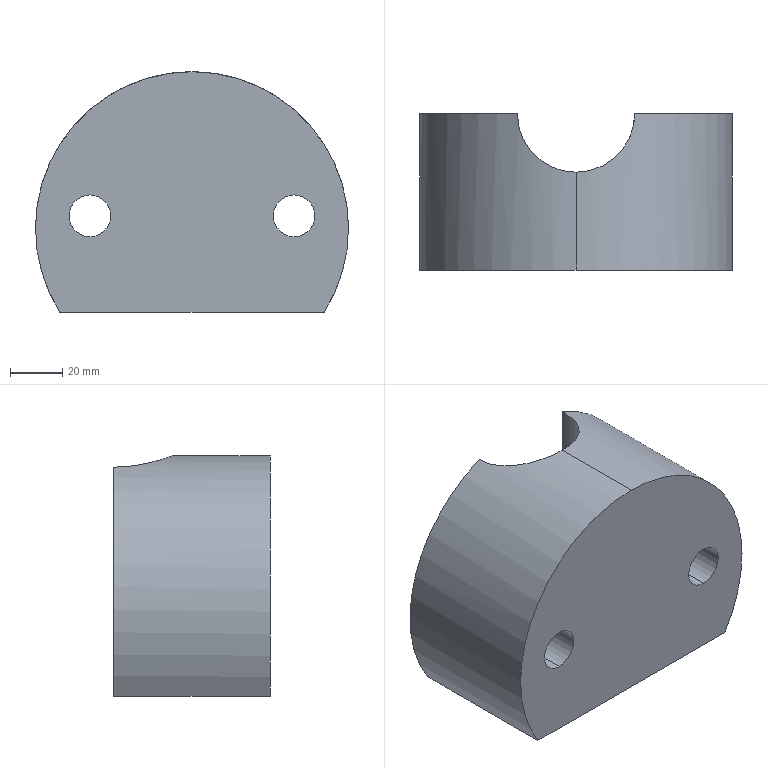Component | SolidWorks | PressureBlock-1 | 1 solid | 12 faces | box 120 x 60 x 92.21 mm | volume 462926 mm3 | cylinder 8 | plane 4 | commonest cylinder face diameters 16 x4 45 x2 120 x2
build123d program:
from build123d import *

# Parameters (mm, degrees)
BOSS_EXTRUDE1_DEPTH        = 60
M39_CLEARANCE_HOLE1_D      = 45
F_16_0_16_DIAMETER_HOLE1_D = 16


with BuildPart() as part:
    # Sketch1 → Boss-Extrude1 (new body)
    with BuildSketch(Plane.XY.offset(60)):
        with BuildLine():
            Line((-37.256, 16.825), (-37.256, -84.417))
            ThreePointArc((-37.256, -84.417), (54.954, -33.796), (-37.256, 16.825))
        make_face()
    extrude(amount=-BOSS_EXTRUDE1_DEPTH)

    # M39 Clearance Hole1 (through all)
    with Locations(Plane.ZY.offset(37.256)):
        with Locations((0, -33.796)):
            Hole(M39_CLEARANCE_HOLE1_D / 2)

    # 16.0 _16_ Diameter Hole1 (through all)
    with Locations(Plane(origin=(0, 0, 0), x_dir=(-1, 0, 0), z_dir=(0, 0, -1))):
        with Locations((0.3007, -72.931), (0.3007, 5.34)):
            Hole(F_16_0_16_DIAMETER_HOLE1_D / 2)


solid = part.part

# Placed as in the assembly
solid = solid.moved(Location((-536.128, 847.548, 422.709), (90, 0, 90)))
STEP:
#1=COLOUR_RGB('',0.7922,0.8196,0.9333);
#2=FILL_AREA_STYLE_COLOUR('',#1);
#3=FILL_AREA_STYLE('',(#2));
#4=SURFACE_STYLE_FILL_AREA(#3);
#5=SURFACE_SIDE_STYLE('',(#4));
#6=SURFACE_STYLE_USAGE(.BOTH.,#5);
#7=PRESENTATION_STYLE_ASSIGNMENT((#6));
#8=CARTESIAN_POINT('',(-18.236,31.006,16.945));
#9=VERTEX_POINT('',#8);
#10=CARTESIAN_POINT('',(-18.236,31.006,16.315));
#11=VERTEX_POINT('',#10);
#12=CARTESIAN_POINT('',(-18.236,31.006,16.63));
#13=DIRECTION('',(0.,1.,0.));
#14=DIRECTION('',(0.,0.,-1.));
#15=AXIS2_PLACEMENT_3D('',#12,#13,#14);
#16=CIRCLE('',#15,0.315);
#17=EDGE_CURVE('',#9,#11,#16,.T.);
#18=ORIENTED_EDGE('',*,*,#17,.F.);
#19=CARTESIAN_POINT('',(-18.236,33.368,16.945));
#20=VERTEX_POINT('',#19);
#21=CARTESIAN_POINT('',(-18.236,33.368,16.945));
#22=DIRECTION('',(0.,1.,0.));
#23=VECTOR('',#22,39.37);
#24=LINE('',#21,#23);
#25=EDGE_CURVE('',#9,#20,#24,.T.);
#26=ORIENTED_EDGE('',*,*,#25,.T.);
#27=CARTESIAN_POINT('',(-18.236,33.368,16.315));
#28=VERTEX_POINT('',#27);
#29=CARTESIAN_POINT('',(-18.236,33.368,16.63));
#30=DIRECTION('',(0.,1.,0.));
#31=DIRECTION('',(0.,0.,-1.));
#32=AXIS2_PLACEMENT_3D('',#29,#30,#31);
#33=CIRCLE('',#32,0.315);
#34=EDGE_CURVE('',#20,#28,#33,.T.);
#35=ORIENTED_EDGE('',*,*,#34,.T.);
#36=CARTESIAN_POINT('',(-18.236,33.368,16.315));
#37=DIRECTION('',(0.,1.,0.));
#38=VECTOR('',#37,39.37);
#39=LINE('',#36,#38);
#40=EDGE_CURVE('',#11,#28,#39,.T.);
#41=ORIENTED_EDGE('',*,*,#40,.F.);
#42=EDGE_LOOP('',(#18,#26,#35,#41));
#43=FACE_OUTER_BOUND('',#42,.T.);
#44=CARTESIAN_POINT('',(-18.236,33.368,16.63));
#45=DIRECTION('',(0.,1.,0.));
#46=DIRECTION('',(0.,0.,-1.));
#47=AXIS2_PLACEMENT_3D('',#44,#45,#46);
#48=CYLINDRICAL_SURFACE('',#47,0.315);
#49=ADVANCED_FACE('',(#43),#48,.F.);
#50=CARTESIAN_POINT('',(-21.318,31.006,16.945));
#51=VERTEX_POINT('',#50);
#52=CARTESIAN_POINT('',(-21.318,31.006,16.315));
#53=VERTEX_POINT('',#52);
#54=CARTESIAN_POINT('',(-21.318,31.006,16.63));
#55=DIRECTION('',(0.,1.,0.));
#56=DIRECTION('',(0.,0.,-1.));
#57=AXIS2_PLACEMENT_3D('',#54,#55,#56);
#58=CIRCLE('',#57,0.315);
#59=EDGE_CURVE('',#51,#53,#58,.T.);
#60=ORIENTED_EDGE('',*,*,#59,.F.);
#61=CARTESIAN_POINT('',(-21.318,33.368,16.945));
#62=VERTEX_POINT('',#61);
#63=CARTESIAN_POINT('',(-21.318,33.368,16.945));
#64=DIRECTION('',(0.,1.,0.));
#65=VECTOR('',#64,39.37);
#66=LINE('',#63,#65);
#67=EDGE_CURVE('',#51,#62,#66,.T.);
#68=ORIENTED_EDGE('',*,*,#67,.T.);
#69=CARTESIAN_POINT('',(-21.318,33.368,16.315));
#70=VERTEX_POINT('',#69);
#71=CARTESIAN_POINT('',(-21.318,33.368,16.63));
#72=DIRECTION('',(0.,1.,0.));
#73=DIRECTION('',(0.,0.,-1.));
#74=AXIS2_PLACEMENT_3D('',#71,#72,#73);
#75=CIRCLE('',#74,0.315);
#76=EDGE_CURVE('',#62,#70,#75,.T.);
#77=ORIENTED_EDGE('',*,*,#76,.T.);
#78=CARTESIAN_POINT('',(-21.318,33.368,16.315));
#79=DIRECTION('',(0.,1.,0.));
#80=VECTOR('',#79,39.37);
#81=LINE('',#78,#80);
#82=EDGE_CURVE('',#53,#70,#81,.T.);
#83=ORIENTED_EDGE('',*,*,#82,.F.);
#84=EDGE_LOOP('',(#60,#68,#77,#83));
#85=FACE_OUTER_BOUND('',#84,.T.);
#86=CARTESIAN_POINT('',(-21.318,33.368,16.63));
#87=DIRECTION('',(0.,1.,0.));
#88=DIRECTION('',(0.,0.,-1.));
#89=AXIS2_PLACEMENT_3D('',#86,#87,#88);
#90=CYLINDRICAL_SURFACE('',#89,0.315);
#91=ADVANCED_FACE('',(#85),#90,.F.);
#92=CARTESIAN_POINT('',(-20.663,33.368,18.633));
#93=VERTEX_POINT('',#92);
#94=CARTESIAN_POINT('',(-19.777,32.482,18.806));
#95=VERTEX_POINT('',#94);
#96=CARTESIAN_POINT('',(-20.663,33.368,18.633));
#97=CARTESIAN_POINT('',(-20.663,33.309,18.633));
#98=CARTESIAN_POINT('',(-20.657,33.251,18.636));
#99=CARTESIAN_POINT('',(-20.64,33.166,18.642));
#100=CARTESIAN_POINT('',(-20.633,33.137,18.645));
#101=CARTESIAN_POINT('',(-20.62,33.095,18.65));
#102=CARTESIAN_POINT('',(-20.615,33.082,18.652));
#103=CARTESIAN_POINT('',(-20.605,33.054,18.656));
#104=CARTESIAN_POINT('',(-20.6,33.041,18.658));
#105=CARTESIAN_POINT('',(-20.572,32.974,18.668));
#106=CARTESIAN_POINT('',(-20.545,32.923,18.678));
#107=CARTESIAN_POINT('',(-20.497,32.851,18.693));
#108=CARTESIAN_POINT('',(-20.479,32.828,18.699));
#109=CARTESIAN_POINT('',(-20.443,32.783,18.71));
#110=CARTESIAN_POINT('',(-20.424,32.762,18.715));
#111=CARTESIAN_POINT('',(-20.383,32.722,18.727));
#112=CARTESIAN_POINT('',(-20.362,32.702,18.732));
#113=CARTESIAN_POINT('',(-20.318,32.666,18.743));
#114=CARTESIAN_POINT('',(-20.295,32.649,18.748));
#115=CARTESIAN_POINT('',(-20.222,32.6,18.764));
#116=CARTESIAN_POINT('',(-20.172,32.573,18.773));
#117=CARTESIAN_POINT('',(-20.092,32.54,18.785));
#118=CARTESIAN_POINT('',(-20.065,32.53,18.788));
#119=CARTESIAN_POINT('',(-20.009,32.513,18.794));
#120=CARTESIAN_POINT('',(-19.98,32.505,18.797));
#121=CARTESIAN_POINT('',(-19.894,32.488,18.803));
#122=CARTESIAN_POINT('',(-19.836,32.482,18.806));
#123=CARTESIAN_POINT('',(-19.777,32.482,18.806));
#124=B_SPLINE_CURVE_WITH_KNOTS('',3,(#96,#97,#98,#99,#100,#101,#102,#103,#104,#105,#106,#107,#108,#109,#110,#111,#112,#113,#114,#115,#116,#117,#118,#119,#120,#121,#122,#123),.UNSPECIFIED.,.F.,.F.,(4,2,2,2,2,2,2,2,2,2,2,2,2,4),(-0.03548,-0.03104,-0.02883,-0.02772,-0.02661,-0.02217,-0.01996,-0.01774,-0.01552,-0.0133,-0.00887,-0.006652,-0.004435,-0.),.UNSPECIFIED.);
#125=EDGE_CURVE('',#93,#95,#124,.T.);
#126=ORIENTED_EDGE('',*,*,#125,.T.);
#127=CARTESIAN_POINT('',(-19.777,32.482,15.175));
#128=VERTEX_POINT('',#127);
#129=CARTESIAN_POINT('',(-19.777,32.482,15.175));
#130=DIRECTION('',(0.,0.,-1.));
#131=VECTOR('',#130,39.37);
#132=LINE('',#129,#131);
#133=EDGE_CURVE('',#95,#128,#132,.T.);
#134=ORIENTED_EDGE('',*,*,#133,.T.);
#135=CARTESIAN_POINT('',(-20.663,33.368,15.175));
#136=VERTEX_POINT('',#135);
#137=CARTESIAN_POINT('',(-19.777,33.368,15.175));
#138=DIRECTION('',(0.,0.,-1.));
#139=DIRECTION('',(0.,-1.,0.));
#140=AXIS2_PLACEMENT_3D('',#137,#138,#139);
#141=CIRCLE('',#140,0.8858);
#142=EDGE_CURVE('',#128,#136,#141,.T.);
#143=ORIENTED_EDGE('',*,*,#142,.T.);
#144=CARTESIAN_POINT('',(-20.663,33.368,15.175));
#145=DIRECTION('',(0.,0.,-1.));
#146=VECTOR('',#145,39.37);
#147=LINE('',#144,#146);
#148=EDGE_CURVE('',#93,#136,#147,.T.);
#149=ORIENTED_EDGE('',*,*,#148,.F.);
#150=EDGE_LOOP('',(#126,#134,#143,#149));
#151=FACE_OUTER_BOUND('',#150,.T.);
#152=CARTESIAN_POINT('',(-19.777,33.368,15.175));
#153=DIRECTION('',(0.,0.,-1.));
#154=DIRECTION('',(0.,-1.,0.));
#155=AXIS2_PLACEMENT_3D('',#152,#153,#154);
#156=CYLINDRICAL_SURFACE('',#155,0.8858);
#157=ADVANCED_FACE('',(#151),#156,.F.);
#158=CARTESIAN_POINT('',(-18.891,33.368,18.633));
#159=VERTEX_POINT('',#158);
#160=CARTESIAN_POINT('',(-19.777,32.482,18.806));
#161=CARTESIAN_POINT('',(-19.718,32.482,18.806));
#162=CARTESIAN_POINT('',(-19.66,32.488,18.803));
#163=CARTESIAN_POINT('',(-19.574,32.505,18.797));
#164=CARTESIAN_POINT('',(-19.546,32.512,18.795));
#165=CARTESIAN_POINT('',(-19.504,32.525,18.79));
#166=CARTESIAN_POINT('',(-19.49,32.53,18.788));
#167=CARTESIAN_POINT('',(-19.463,32.54,18.785));
#168=CARTESIAN_POINT('',(-19.449,32.545,18.783));
#169=CARTESIAN_POINT('',(-19.382,32.573,18.773));
#170=CARTESIAN_POINT('',(-19.332,32.6,18.764));
#171=CARTESIAN_POINT('',(-19.26,32.648,18.748));
#172=CARTESIAN_POINT('',(-19.236,32.666,18.743));
#173=CARTESIAN_POINT('',(-19.192,32.702,18.732));
#174=CARTESIAN_POINT('',(-19.171,32.721,18.727));
#175=CARTESIAN_POINT('',(-19.11,32.782,18.71));
#176=CARTESIAN_POINT('',(-19.073,32.826,18.699));
#177=CARTESIAN_POINT('',(-19.009,32.923,18.678));
#178=CARTESIAN_POINT('',(-18.982,32.973,18.668));
#179=CARTESIAN_POINT('',(-18.948,33.053,18.656));
#180=CARTESIAN_POINT('',(-18.939,33.08,18.652));
#181=CARTESIAN_POINT('',(-18.921,33.136,18.645));
#182=CARTESIAN_POINT('',(-18.914,33.165,18.643));
#183=CARTESIAN_POINT('',(-18.897,33.251,18.636));
#184=CARTESIAN_POINT('',(-18.891,33.309,18.633));
#185=CARTESIAN_POINT('',(-18.891,33.368,18.633));
#186=B_SPLINE_CURVE_WITH_KNOTS('',3,(#160,#161,#162,#163,#164,#165,#166,#167,#168,#169,#170,#171,#172,#173,#174,#175,#176,#177,#178,#179,#180,#181,#182,#183,#184,#185),.UNSPECIFIED.,.F.,.F.,(4,2,2,2,2,2,2,2,2,2,2,2,4),(-0.,0.004435,0.006652,0.007761,0.00887,0.0133,0.01552,0.01774,0.02217,0.02661,0.02883,0.03104,0.03548),.UNSPECIFIED.);
#187=EDGE_CURVE('',#95,#159,#186,.T.);
#188=ORIENTED_EDGE('',*,*,#187,.F.);
#189=CARTESIAN_POINT('',(-19.777,31.006,18.806));
#190=VERTEX_POINT('',#189);
#191=CARTESIAN_POINT('',(-19.777,33.368,18.806));
#192=DIRECTION('',(0.,-1.,0.));
#193=VECTOR('',#192,39.37);
#194=LINE('',#191,#193);
#195=EDGE_CURVE('',#95,#190,#194,.T.);
#196=ORIENTED_EDGE('',*,*,#195,.T.);
#197=CARTESIAN_POINT('',(-17.784,31.006,15.175));
#198=VERTEX_POINT('',#197);
#199=CARTESIAN_POINT('',(-19.777,31.006,16.443));
#200=DIRECTION('',(0.,-1.,0.));
#201=DIRECTION('',(0.,0.,1.));
#202=AXIS2_PLACEMENT_3D('',#199,#200,#201);
#203=CIRCLE('',#202,2.362);
#204=EDGE_CURVE('',#198,#190,#203,.T.);
#205=ORIENTED_EDGE('',*,*,#204,.F.);
#206=CARTESIAN_POINT('',(-17.784,33.368,15.175));
#207=VERTEX_POINT('',#206);
#208=CARTESIAN_POINT('',(-17.784,33.368,15.175));
#209=DIRECTION('',(0.,-1.,0.));
#210=VECTOR('',#209,39.37);
#211=LINE('',#208,#210);
#212=EDGE_CURVE('',#207,#198,#211,.T.);
#213=ORIENTED_EDGE('',*,*,#212,.F.);
#214=CARTESIAN_POINT('',(-19.777,33.368,16.443));
#215=DIRECTION('',(0.,-1.,0.));
#216=DIRECTION('',(0.,0.,1.));
#217=AXIS2_PLACEMENT_3D('',#214,#215,#216);
#218=CIRCLE('',#217,2.362);
#219=EDGE_CURVE('',#207,#159,#218,.T.);
#220=ORIENTED_EDGE('',*,*,#219,.T.);
#221=EDGE_LOOP('',(#188,#196,#205,#213,#220));
#222=FACE_OUTER_BOUND('',#221,.T.);
#223=CARTESIAN_POINT('',(-19.777,33.368,16.443));
#224=DIRECTION('',(0.,-1.,0.));
#225=DIRECTION('',(0.,0.,1.));
#226=AXIS2_PLACEMENT_3D('',#223,#224,#225);
#227=CYLINDRICAL_SURFACE('',#226,2.362);
#228=ADVANCED_FACE('',(#222),#227,.T.);
#229=ORIENTED_EDGE('',*,*,#204,.T.);
#230=CARTESIAN_POINT('',(-21.77,31.006,15.175));
#231=VERTEX_POINT('',#230);
#232=CARTESIAN_POINT('',(-19.777,31.006,16.443));
#233=DIRECTION('',(0.,-1.,0.));
#234=DIRECTION('',(0.,0.,1.));
#235=AXIS2_PLACEMENT_3D('',#232,#233,#234);
#236=CIRCLE('',#235,2.362);
#237=EDGE_CURVE('',#190,#231,#236,.T.);
#238=ORIENTED_EDGE('',*,*,#237,.T.);
#239=CARTESIAN_POINT('',(-21.77,31.006,15.175));
#240=DIRECTION('',(1.,0.,-0.));
#241=VECTOR('',#240,39.37);
#242=LINE('',#239,#241);
#243=EDGE_CURVE('',#231,#198,#242,.T.);
#244=ORIENTED_EDGE('',*,*,#243,.T.);
#245=EDGE_LOOP('',(#229,#238,#244));
#246=FACE_OUTER_BOUND('',#245,.T.);
#247=CARTESIAN_POINT('',(-21.318,31.006,16.63));
#248=DIRECTION('',(0.,1.,0.));
#249=DIRECTION('',(0.,0.,-1.));
#250=AXIS2_PLACEMENT_3D('',#247,#248,#249);
#251=CIRCLE('',#250,0.315);
#252=EDGE_CURVE('',#53,#51,#251,.T.);
#253=ORIENTED_EDGE('',*,*,#252,.T.);
#254=ORIENTED_EDGE('',*,*,#59,.T.);
#255=EDGE_LOOP('',(#253,#254));
#256=FACE_BOUND('',#255,.T.);
#257=CARTESIAN_POINT('',(-18.236,31.006,16.63));
#258=DIRECTION('',(0.,1.,0.));
#259=DIRECTION('',(0.,0.,-1.));
#260=AXIS2_PLACEMENT_3D('',#257,#258,#259);
#261=CIRCLE('',#260,0.315);
#262=EDGE_CURVE('',#11,#9,#261,.T.);
#263=ORIENTED_EDGE('',*,*,#262,.T.);
#264=ORIENTED_EDGE('',*,*,#17,.T.);
#265=EDGE_LOOP('',(#263,#264));
#266=FACE_BOUND('',#265,.T.);
#267=CARTESIAN_POINT('',(-19.777,31.006,16.443));
#268=DIRECTION('',(0.,-1.,0.));
#269=DIRECTION('',(0.,0.,1.));
#270=AXIS2_PLACEMENT_3D('',#267,#268,#269);
#271=PLANE('',#270);
#272=ADVANCED_FACE('',(#246,#256,#266),#271,.T.);
#273=CARTESIAN_POINT('',(-21.77,33.368,15.175));
#274=VERTEX_POINT('',#273);
#275=CARTESIAN_POINT('',(-19.777,33.368,16.443));
#276=DIRECTION('',(0.,-1.,0.));
#277=DIRECTION('',(0.,0.,1.));
#278=AXIS2_PLACEMENT_3D('',#275,#276,#277);
#279=CIRCLE('',#278,2.362);
#280=EDGE_CURVE('',#93,#274,#279,.T.);
#281=ORIENTED_EDGE('',*,*,#280,.F.);
#282=ORIENTED_EDGE('',*,*,#148,.T.);
#283=CARTESIAN_POINT('',(-21.77,33.368,15.175));
#284=DIRECTION('',(1.,0.,-0.));
#285=VECTOR('',#284,39.37);
#286=LINE('',#283,#285);
#287=EDGE_CURVE('',#274,#136,#286,.T.);
#288=ORIENTED_EDGE('',*,*,#287,.F.);
#289=EDGE_LOOP('',(#281,#282,#288));
#290=FACE_OUTER_BOUND('',#289,.T.);
#291=CARTESIAN_POINT('',(-21.318,33.368,16.63));
#292=DIRECTION('',(0.,1.,0.));
#293=DIRECTION('',(0.,0.,-1.));
#294=AXIS2_PLACEMENT_3D('',#291,#292,#293);
#295=CIRCLE('',#294,0.315);
#296=EDGE_CURVE('',#70,#62,#295,.T.);
#297=ORIENTED_EDGE('',*,*,#296,.F.);
#298=ORIENTED_EDGE('',*,*,#76,.F.);
#299=EDGE_LOOP('',(#297,#298));
#300=FACE_BOUND('',#299,.T.);
#301=CARTESIAN_POINT('',(-19.777,33.368,16.443));
#302=DIRECTION('',(0.,-1.,0.));
#303=DIRECTION('',(0.,0.,1.));
#304=AXIS2_PLACEMENT_3D('',#301,#302,#303);
#305=PLANE('',#304);
#306=ADVANCED_FACE('',(#290,#300),#305,.F.);
#307=ORIENTED_EDGE('',*,*,#195,.F.);
#308=ORIENTED_EDGE('',*,*,#125,.F.);
#309=ORIENTED_EDGE('',*,*,#280,.T.);
#310=CARTESIAN_POINT('',(-21.77,33.368,15.175));
#311=DIRECTION('',(0.,-1.,0.));
#312=VECTOR('',#311,39.37);
#313=LINE('',#310,#312);
#314=EDGE_CURVE('',#274,#231,#313,.T.);
#315=ORIENTED_EDGE('',*,*,#314,.T.);
#316=ORIENTED_EDGE('',*,*,#237,.F.);
#317=EDGE_LOOP('',(#307,#308,#309,#315,#316));
#318=FACE_OUTER_BOUND('',#317,.T.);
#319=CARTESIAN_POINT('',(-19.777,33.368,16.443));
#320=DIRECTION('',(0.,-1.,0.));
#321=DIRECTION('',(0.,0.,1.));
#322=AXIS2_PLACEMENT_3D('',#319,#320,#321);
#323=CYLINDRICAL_SURFACE('',#322,2.362);
#324=ADVANCED_FACE('',(#318),#323,.T.);
#325=CARTESIAN_POINT('',(-18.891,33.368,15.175));
#326=VERTEX_POINT('',#325);
#327=CARTESIAN_POINT('',(-19.777,33.368,15.175));
#328=DIRECTION('',(0.,0.,-1.));
#329=DIRECTION('',(0.,-1.,0.));
#330=AXIS2_PLACEMENT_3D('',#327,#328,#329);
#331=CIRCLE('',#330,0.8858);
#332=EDGE_CURVE('',#326,#128,#331,.T.);
#333=ORIENTED_EDGE('',*,*,#332,.F.);
#334=CARTESIAN_POINT('',(-21.77,33.368,15.175));
#335=DIRECTION('',(1.,0.,-0.));
#336=VECTOR('',#335,39.37);
#337=LINE('',#334,#336);
#338=EDGE_CURVE('',#326,#207,#337,.T.);
#339=ORIENTED_EDGE('',*,*,#338,.T.);
#340=ORIENTED_EDGE('',*,*,#212,.T.);
#341=ORIENTED_EDGE('',*,*,#243,.F.);
#342=ORIENTED_EDGE('',*,*,#314,.F.);
#343=ORIENTED_EDGE('',*,*,#287,.T.);
#344=ORIENTED_EDGE('',*,*,#142,.F.);
#345=EDGE_LOOP('',(#333,#339,#340,#341,#342,#343,#344));
#346=FACE_OUTER_BOUND('',#345,.T.);
#347=CARTESIAN_POINT('',(-21.77,33.368,15.175));
#348=DIRECTION('',(-0.,0.,-1.));
#349=DIRECTION('',(1.,0.,-0.));
#350=AXIS2_PLACEMENT_3D('',#347,#348,#349);
#351=PLANE('',#350);
#352=ADVANCED_FACE('',(#346),#351,.T.);
#353=CARTESIAN_POINT('',(-18.236,33.368,16.63));
#354=DIRECTION('',(0.,1.,0.));
#355=DIRECTION('',(0.,0.,-1.));
#356=AXIS2_PLACEMENT_3D('',#353,#354,#355);
#357=CIRCLE('',#356,0.315);
#358=EDGE_CURVE('',#28,#20,#357,.T.);
#359=ORIENTED_EDGE('',*,*,#358,.F.);
#360=ORIENTED_EDGE('',*,*,#34,.F.);
#361=EDGE_LOOP('',(#359,#360));
#362=FACE_BOUND('',#361,.T.);
#363=ORIENTED_EDGE('',*,*,#338,.F.);
#364=CARTESIAN_POINT('',(-18.891,33.368,15.175));
#365=DIRECTION('',(0.,0.,1.));
#366=VECTOR('',#365,39.37);
#367=LINE('',#364,#366);
#368=EDGE_CURVE('',#326,#159,#367,.T.);
#369=ORIENTED_EDGE('',*,*,#368,.T.);
#370=ORIENTED_EDGE('',*,*,#219,.F.);
#371=EDGE_LOOP('',(#363,#369,#370));
#372=FACE_OUTER_BOUND('',#371,.T.);
#373=CARTESIAN_POINT('',(-19.777,33.368,16.443));
#374=DIRECTION('',(0.,-1.,0.));
#375=DIRECTION('',(0.,0.,1.));
#376=AXIS2_PLACEMENT_3D('',#373,#374,#375);
#377=PLANE('',#376);
#378=ADVANCED_FACE('',(#362,#372),#377,.F.);
#379=ORIENTED_EDGE('',*,*,#133,.F.);
#380=ORIENTED_EDGE('',*,*,#187,.T.);
#381=ORIENTED_EDGE('',*,*,#368,.F.);
#382=ORIENTED_EDGE('',*,*,#332,.T.);
#383=EDGE_LOOP('',(#379,#380,#381,#382));
#384=FACE_OUTER_BOUND('',#383,.T.);
#385=CARTESIAN_POINT('',(-19.777,33.368,15.175));
#386=DIRECTION('',(0.,0.,-1.));
#387=DIRECTION('',(0.,-1.,0.));
#388=AXIS2_PLACEMENT_3D('',#385,#386,#387);
#389=CYLINDRICAL_SURFACE('',#388,0.8858);
#390=ADVANCED_FACE('',(#384),#389,.F.);
#391=ORIENTED_EDGE('',*,*,#67,.F.);
#392=ORIENTED_EDGE('',*,*,#252,.F.);
#393=ORIENTED_EDGE('',*,*,#82,.T.);
#394=ORIENTED_EDGE('',*,*,#296,.T.);
#395=EDGE_LOOP('',(#391,#392,#393,#394));
#396=FACE_OUTER_BOUND('',#395,.T.);
#397=CARTESIAN_POINT('',(-21.318,33.368,16.63));
#398=DIRECTION('',(0.,1.,0.));
#399=DIRECTION('',(0.,0.,-1.));
#400=AXIS2_PLACEMENT_3D('',#397,#398,#399);
#401=CYLINDRICAL_SURFACE('',#400,0.315);
#402=ADVANCED_FACE('',(#396),#401,.F.);
#403=ORIENTED_EDGE('',*,*,#25,.F.);
#404=ORIENTED_EDGE('',*,*,#262,.F.);
#405=ORIENTED_EDGE('',*,*,#40,.T.);
#406=ORIENTED_EDGE('',*,*,#358,.T.);
#407=EDGE_LOOP('',(#403,#404,#405,#406));
#408=FACE_OUTER_BOUND('',#407,.T.);
#409=CARTESIAN_POINT('',(-18.236,33.368,16.63));
#410=DIRECTION('',(0.,1.,0.));
#411=DIRECTION('',(0.,0.,-1.));
#412=AXIS2_PLACEMENT_3D('',#409,#410,#411);
#413=CYLINDRICAL_SURFACE('',#412,0.315);
#414=ADVANCED_FACE('',(#408),#413,.F.);
#415=CLOSED_SHELL('',(#49,#91,#157,#228,#272,#306,#324,#352,#378,#390,#402,#414));
#416=MANIFOLD_SOLID_BREP('',#415);
#417=STYLED_ITEM('',(#7),#416);
#418=(LENGTH_UNIT()NAMED_UNIT(*)SI_UNIT($,.METRE.));
#419=LENGTH_MEASURE_WITH_UNIT(LENGTH_MEASURE(0.0254),#418);
#420=DIMENSIONAL_EXPONENTS(1.,0.,0.,0.,0.,0.,0.);
#421=(CONVERSION_BASED_UNIT('',#419)LENGTH_UNIT()NAMED_UNIT(#420));
#422=UNCERTAINTY_MEASURE_WITH_UNIT(LENGTH_MEASURE(0.00001),#421,'','');
#423=(NAMED_UNIT(*)PLANE_ANGLE_UNIT()SI_UNIT($,.RADIAN.));
#424=(NAMED_UNIT(*)SI_UNIT($,.STERADIAN.)SOLID_ANGLE_UNIT());
#425=(GEOMETRIC_REPRESENTATION_CONTEXT(3)GLOBAL_UNCERTAINTY_ASSIGNED_CONTEXT((#422))GLOBAL_UNIT_ASSIGNED_CONTEXT((#421,#423,#424))REPRESENTATION_CONTEXT('',''));
#426=MECHANICAL_DESIGN_GEOMETRIC_PRESENTATION_REPRESENTATION('',(#417),#425);
#427=CARTESIAN_POINT('',(0.,0.,0.));
#428=DIRECTION('',(0.,0.,1.));
#429=DIRECTION('',(1.,0.,0.));
#430=AXIS2_PLACEMENT_3D('',#427,#428,#429);
#431=(LENGTH_UNIT()NAMED_UNIT(*)SI_UNIT($,.METRE.));
#432=LENGTH_MEASURE_WITH_UNIT(LENGTH_MEASURE(0.0254),#431);
#433=DIMENSIONAL_EXPONENTS(1.,0.,0.,0.,0.,0.,0.);
#434=(CONVERSION_BASED_UNIT('',#432)LENGTH_UNIT()NAMED_UNIT(#433));
#435=UNCERTAINTY_MEASURE_WITH_UNIT(LENGTH_MEASURE(0.00001),#434,'','');
#436=(NAMED_UNIT(*)PLANE_ANGLE_UNIT()SI_UNIT($,.RADIAN.));
#437=(NAMED_UNIT(*)SI_UNIT($,.STERADIAN.)SOLID_ANGLE_UNIT());
#438=(GEOMETRIC_REPRESENTATION_CONTEXT(3)GLOBAL_UNCERTAINTY_ASSIGNED_CONTEXT((#435))GLOBAL_UNIT_ASSIGNED_CONTEXT((#434,#436,#437))REPRESENTATION_CONTEXT('',''));
#439=ADVANCED_BREP_SHAPE_REPRESENTATION('',(#416,#430),#438);
#440=PRESENTATION_LAYER_ASSIGNMENT('','',(#417));